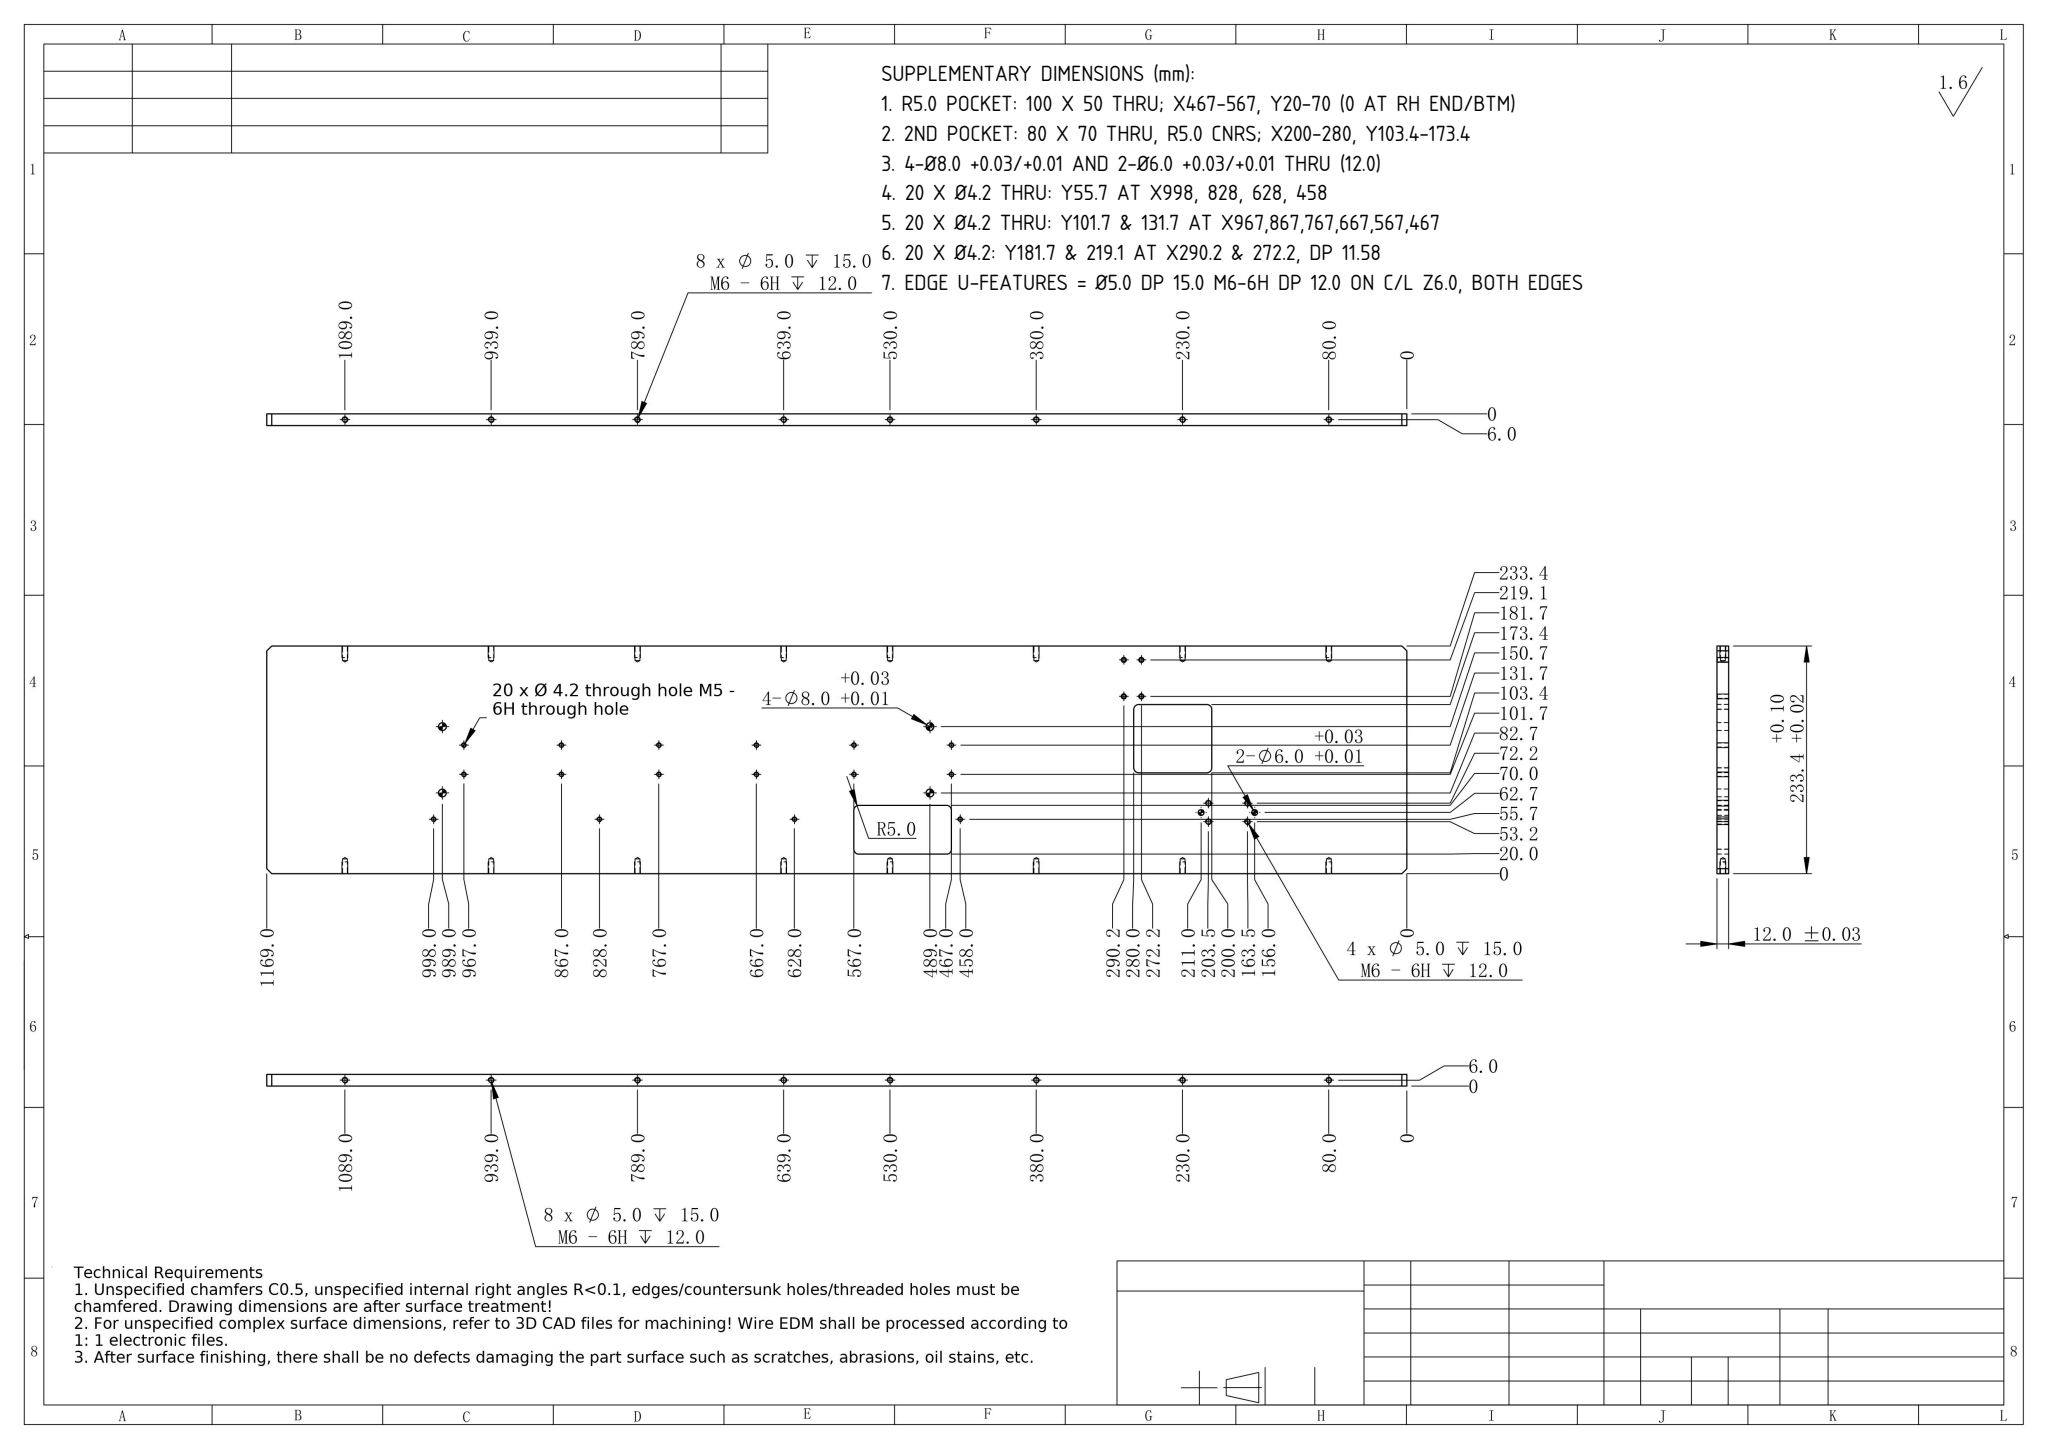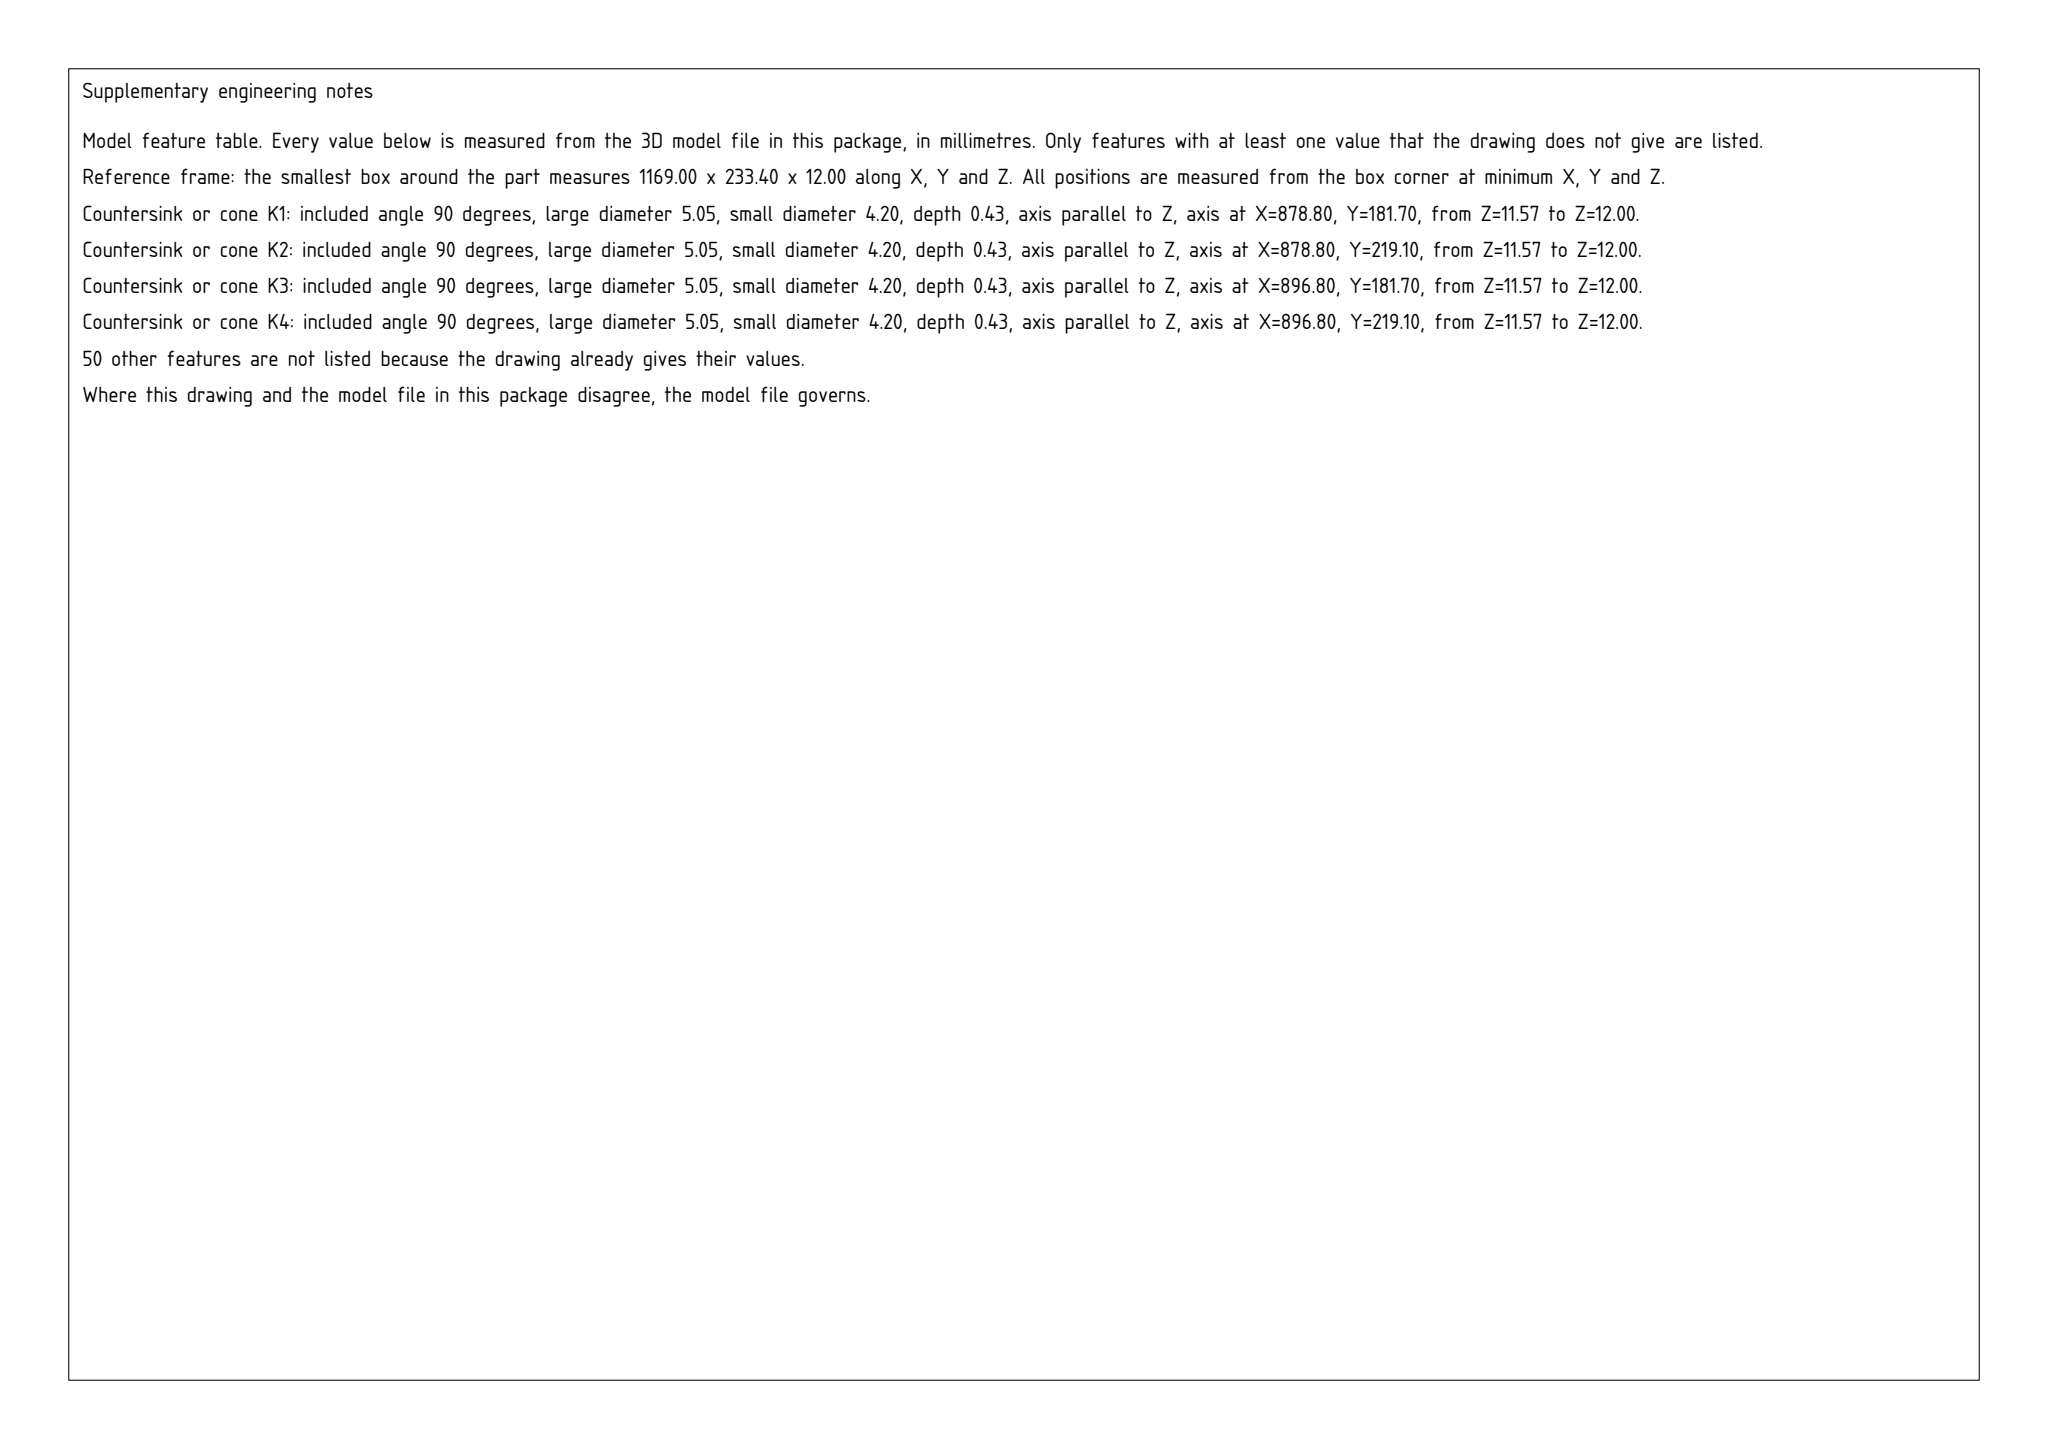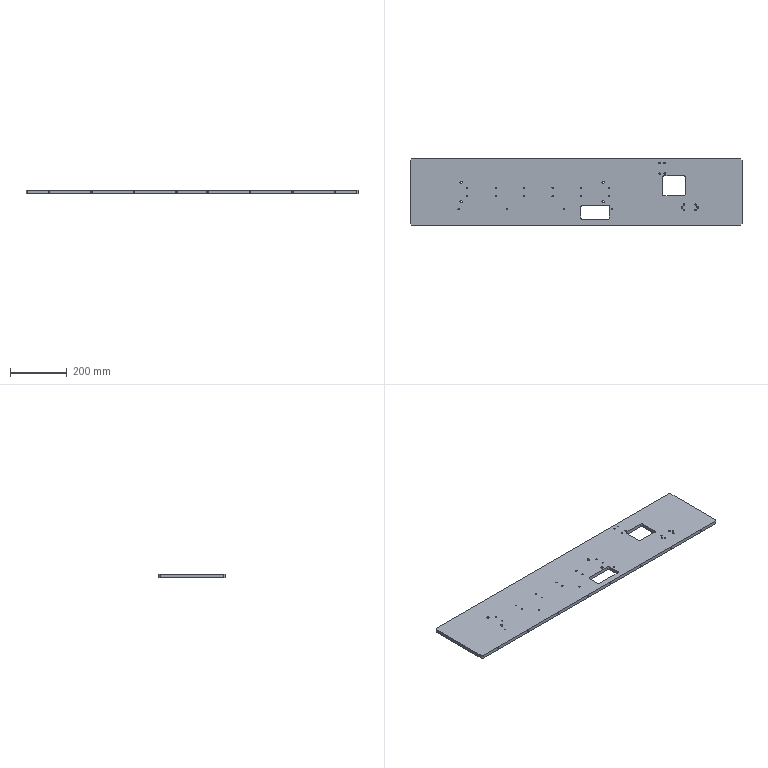Part | SolidWorks | mm | 1 solid | 158 faces | box 1169 x 233.4 x 12 mm | volume 3134617 mm3 | cylinder 100 | cone 40 | plane 18 | commonest cylinder face diameters 5 x40 4.2 x40 8 x8 10 x8 6 x4
build123d program:
from build123d import *

# Parameters (mm, degrees)
SKETCH1_W                   = 1169
SKETCH1_H                   = 233.4
BOSS_EXTRUDE1_DEPTH         = 6
CHAMFER1_SIZE               = 5
M5_TAPPED_HOLE1_D           = 4.2
M5_TAPPED_HOLE2_D           = 4.2
SKETCH8_R                   = 4
CUT_EXTRUDE1_DEPTH          = 20
M5_TAPPED_HOLE3_D           = 4.2
M5_TAPPED_HOLE3_CSINK_D     = 5.05
M5_TAPPED_HOLE3_CSINK_ANGLE = 90
M6_TAPPED_HOLE2_AT_2_COUNT  = 2
M6_TAPPED_HOLE2_AT_2_PITCH  = 150
M6_TAPPED_HOLE2_AT_3_COUNT  = 2
M6_TAPPED_HOLE2_AT_3_PITCH  = 300
M6_TAPPED_HOLE2_AT_4_COUNT  = 2
M6_TAPPED_HOLE2_AT_4_PITCH  = 450
M6_TAPPED_HOLE2_AT_5_COUNT  = 2
M6_TAPPED_HOLE2_AT_5_PITCH  = 559
M6_TAPPED_HOLE2_AT_6_COUNT  = 2
M6_TAPPED_HOLE2_AT_6_PITCH  = 709
M6_TAPPED_HOLE2_AT_7_COUNT  = 2
M6_TAPPED_HOLE2_AT_7_PITCH  = 859
M6_TAPPED_HOLE2_AT_8_COUNT  = 2
M6_TAPPED_HOLE2_AT_8_PITCH  = 1009
M6_TAPPED_HOLE3_D           = 5
M6_TAPPED_HOLE3_DEPTH       = 15
M6_TAPPED_HOLE3_TIP         = 1.502
SKETCH15_R                  = 3
CUT_EXTRUDE2_DEPTH          = 49
SKETCH16_W                  = 80
SKETCH16_H                  = 70
SKETCH16_W_2                = 100
SKETCH16_H_2                = 50
CUT_EXTRUDE3_DEPTH          = 597.157
FILLET1_R                   = 5


with BuildPart() as part:
    # Sketch1 → Boss-Extrude1 (new, symmetric)
    with BuildSketch(Plane.XY):
        Rectangle(SKETCH1_W, SKETCH1_H)
    extrude(amount=BOSS_EXTRUDE1_DEPTH, both=True)

    # Chamfer1
    chamfer1_edges = [part.edges().sort_by_distance(p)[0] for p in [
        (-584.5, 116.7, 0),
        (584.5, 116.7, 0),
        (584.5, -116.7, 0),
        (-584.5, -116.7, 0),
    ]]
    chamfer(chamfer1_edges, length=CHAMFER1_SIZE)

    # M5 Tapped Hole1 (through all)
    with Locations(Plane.XY.offset(6)):
        with Locations((-413.5, -61), (-243.5, -61), (-43.5, -61), (126.5, -61)):
            Hole(M5_TAPPED_HOLE1_D / 2)

    # M5 Tapped Hole2 (through all)
    with Locations(Plane(origin=(0, 0, -6), x_dir=(-1, 0, 0), z_dir=(0, 0, -1))):
        with Locations((-117.5, 15), (-117.5, -15), (-17.5, -15), (-17.5, 15), (82.5, 15), (82.5, -15), (182.5, -15), (182.5, 15), (282.5, 15), (282.5, -15), (382.5, -15), (382.5, 15)):
            Hole(M5_TAPPED_HOLE2_D / 2)

    # Sketch8 → Cut-Extrude1 (cut)
    with BuildSketch(Plane.XY.offset(6)):
        with Locations((-404.5, 34)):
            Circle(SKETCH8_R)
        with Locations((95.5, 34)):
            Circle(SKETCH8_R)
        with Locations((95.5, -34)):
            Circle(SKETCH8_R)
        with Locations((-404.5, -34)):
            Circle(SKETCH8_R)
    extrude(amount=-CUT_EXTRUDE1_DEPTH, mode=Mode.SUBTRACT)

    # M5 Tapped Hole3 (through all)
    with Locations(Plane.XY.offset(6)):
        with Locations((312.3, 65), (312.3, 102.4), (294.3, 102.4), (294.3, 65)):
            CounterSinkHole(M5_TAPPED_HOLE3_D / 2, M5_TAPPED_HOLE3_CSINK_D / 2, counter_sink_angle=M5_TAPPED_HOLE3_CSINK_ANGLE)

    # Sketch12 → M6 Tapped Hole2 (revolve, cut)
    with BuildSketch(Plane(origin=(-504.5, 116.7, 0), x_dir=(0, 0, 1), z_dir=(1, 0, 0))):
        Polygon((0, 0), (0, 16.502), (2.5, 15), (2.5, 0), align=None)
    m6_tapped_hole2 = revolve(axis=Axis((-504.5, 123.05, 0), (0, -1, 0)), mode=Mode.SUBTRACT)

    # M6 Tapped Hole2 at 2: M6 Tapped Hole2 ×2
    with Locations(*[(i * M6_TAPPED_HOLE2_AT_2_PITCH, 0, 0) for i in range(1, M6_TAPPED_HOLE2_AT_2_COUNT)]):
        add(m6_tapped_hole2, mode=Mode.SUBTRACT)

    # M6 Tapped Hole2 at 3: M6 Tapped Hole2 ×2
    with Locations(*[(i * M6_TAPPED_HOLE2_AT_3_PITCH, 0, 0) for i in range(1, M6_TAPPED_HOLE2_AT_3_COUNT)]):
        add(m6_tapped_hole2, mode=Mode.SUBTRACT)

    # M6 Tapped Hole2 at 4: M6 Tapped Hole2 ×2
    with Locations(*[(i * M6_TAPPED_HOLE2_AT_4_PITCH, 0, 0) for i in range(1, M6_TAPPED_HOLE2_AT_4_COUNT)]):
        add(m6_tapped_hole2, mode=Mode.SUBTRACT)

    # M6 Tapped Hole2 at 5: M6 Tapped Hole2 ×2
    with Locations(*[(i * M6_TAPPED_HOLE2_AT_5_PITCH, 0, 0) for i in range(1, M6_TAPPED_HOLE2_AT_5_COUNT)]):
        add(m6_tapped_hole2, mode=Mode.SUBTRACT)

    # M6 Tapped Hole2 at 6: M6 Tapped Hole2 ×2
    with Locations(*[(i * M6_TAPPED_HOLE2_AT_6_PITCH, 0, 0) for i in range(1, M6_TAPPED_HOLE2_AT_6_COUNT)]):
        add(m6_tapped_hole2, mode=Mode.SUBTRACT)

    # M6 Tapped Hole2 at 7: M6 Tapped Hole2 ×2
    with Locations(*[(i * M6_TAPPED_HOLE2_AT_7_PITCH, 0, 0) for i in range(1, M6_TAPPED_HOLE2_AT_7_COUNT)]):
        add(m6_tapped_hole2, mode=Mode.SUBTRACT)

    # M6 Tapped Hole2 at 8: M6 Tapped Hole2 ×2
    with Locations(*[(i * M6_TAPPED_HOLE2_AT_8_PITCH, 0, 0) for i in range(1, M6_TAPPED_HOLE2_AT_8_COUNT)]):
        add(m6_tapped_hole2, mode=Mode.SUBTRACT)

    # Mirror1: M6 Tapped Hole2 across plane
    add(m6_tapped_hole2.mirror(Plane.ZX), mode=Mode.SUBTRACT)

    # Mirror1 copy 1 sketch → Mirror1 copy 1 (revolve, cut)
    with BuildSketch(Plane(origin=(-354.5, -116.7, 0), x_dir=(0, 0, 1), z_dir=(1, 0, 0))):
        Polygon((0, 0), (0, -16.502), (2.5, -15), (2.5, 0), align=None)
    revolve(axis=Axis((-354.5, -123.05, 0), (0, -1, 0)), mode=Mode.SUBTRACT)

    # Mirror1 copy 2 sketch → Mirror1 copy 2 (revolve, cut)
    with BuildSketch(Plane(origin=(-204.5, -116.7, 0), x_dir=(0, 0, 1), z_dir=(1, 0, 0))):
        Polygon((0, 0), (0, -16.502), (2.5, -15), (2.5, 0), align=None)
    revolve(axis=Axis((-204.5, -123.05, 0), (0, -1, 0)), mode=Mode.SUBTRACT)

    # Mirror1 copy 3 sketch → Mirror1 copy 3 (revolve, cut)
    with BuildSketch(Plane(origin=(-54.5, -116.7, 0), x_dir=(0, 0, 1), z_dir=(1, 0, 0))):
        Polygon((0, 0), (0, -16.502), (2.5, -15), (2.5, 0), align=None)
    revolve(axis=Axis((-54.5, -123.05, 0), (0, -1, 0)), mode=Mode.SUBTRACT)

    # Mirror1 copy 4 sketch → Mirror1 copy 4 (revolve, cut)
    with BuildSketch(Plane(origin=(54.5, -116.7, 0), x_dir=(0, 0, 1), z_dir=(1, 0, 0))):
        Polygon((0, 0), (0, -16.502), (2.5, -15), (2.5, 0), align=None)
    revolve(axis=Axis((54.5, -123.05, 0), (0, -1, 0)), mode=Mode.SUBTRACT)

    # Mirror1 copy 5 sketch → Mirror1 copy 5 (revolve, cut)
    with BuildSketch(Plane(origin=(204.5, -116.7, 0), x_dir=(0, 0, 1), z_dir=(1, 0, 0))):
        Polygon((0, 0), (0, -16.502), (2.5, -15), (2.5, 0), align=None)
    revolve(axis=Axis((204.5, -123.05, 0), (0, -1, 0)), mode=Mode.SUBTRACT)

    # Mirror1 copy 6 sketch → Mirror1 copy 6 (revolve, cut)
    with BuildSketch(Plane(origin=(354.5, -116.7, 0), x_dir=(0, 0, 1), z_dir=(1, 0, 0))):
        Polygon((0, 0), (0, -16.502), (2.5, -15), (2.5, 0), align=None)
    revolve(axis=Axis((354.5, -123.05, 0), (0, -1, 0)), mode=Mode.SUBTRACT)

    # Mirror1 copy 7 sketch → Mirror1 copy 7 (revolve, cut)
    with BuildSketch(Plane(origin=(504.5, -116.7, 0), x_dir=(0, 0, 1), z_dir=(1, 0, 0))):
        Polygon((0, 0), (0, -16.502), (2.5, -15), (2.5, 0), align=None)
    revolve(axis=Axis((504.5, -123.05, 0), (0, -1, 0)), mode=Mode.SUBTRACT)

    # M6 Tapped Hole3
    with Locations(Plane.XY.offset(6)):
        with Locations((421, -44.5), (381, -44.5), (381, -63.5), (421, -63.5)):
            Hole(M6_TAPPED_HOLE3_D / 2, depth=M6_TAPPED_HOLE3_DEPTH)
            with Locations((0, 0, -(M6_TAPPED_HOLE3_DEPTH + M6_TAPPED_HOLE3_TIP / 2))):  # 118° drill point
                Cone(0, M6_TAPPED_HOLE3_D / 2, M6_TAPPED_HOLE3_TIP, mode=Mode.SUBTRACT)

    # Sketch15 → Cut-Extrude2 (cut)
    with BuildSketch(Plane.XY.offset(6)):
        with Locations((428.5, -54)):
            Circle(SKETCH15_R)
        with Locations((373.5, -54)):
            Circle(SKETCH15_R)
    extrude(amount=-CUT_EXTRUDE2_DEPTH, mode=Mode.SUBTRACT)

    # Sketch16 → Cut-Extrude3 (cut, through all)
    with BuildSketch(Plane.XY.offset(6)):
        with Locations((344.5, 21.7)):
            Rectangle(SKETCH16_W, SKETCH16_H)
        with Locations((67.5, -71.7)):
            Rectangle(SKETCH16_W_2, SKETCH16_H_2)
    extrude(amount=-CUT_EXTRUDE3_DEPTH, mode=Mode.SUBTRACT)

    # Fillet1
    fillet1_edges = [part.edges().sort_by_distance(p)[0] for p in [
        (304.5, -13.3, 0),
        (304.5, 56.7, 0),
        (384.5, 56.7, 0),
        (384.5, -13.3, 0),
        (17.5, -96.7, 0),
        (17.5, -46.7, 0),
        (117.5, -46.7, 0),
        (117.5, -96.7, 0),
    ]]
    fillet(fillet1_edges, radius=FILLET1_R)


solid = part.part